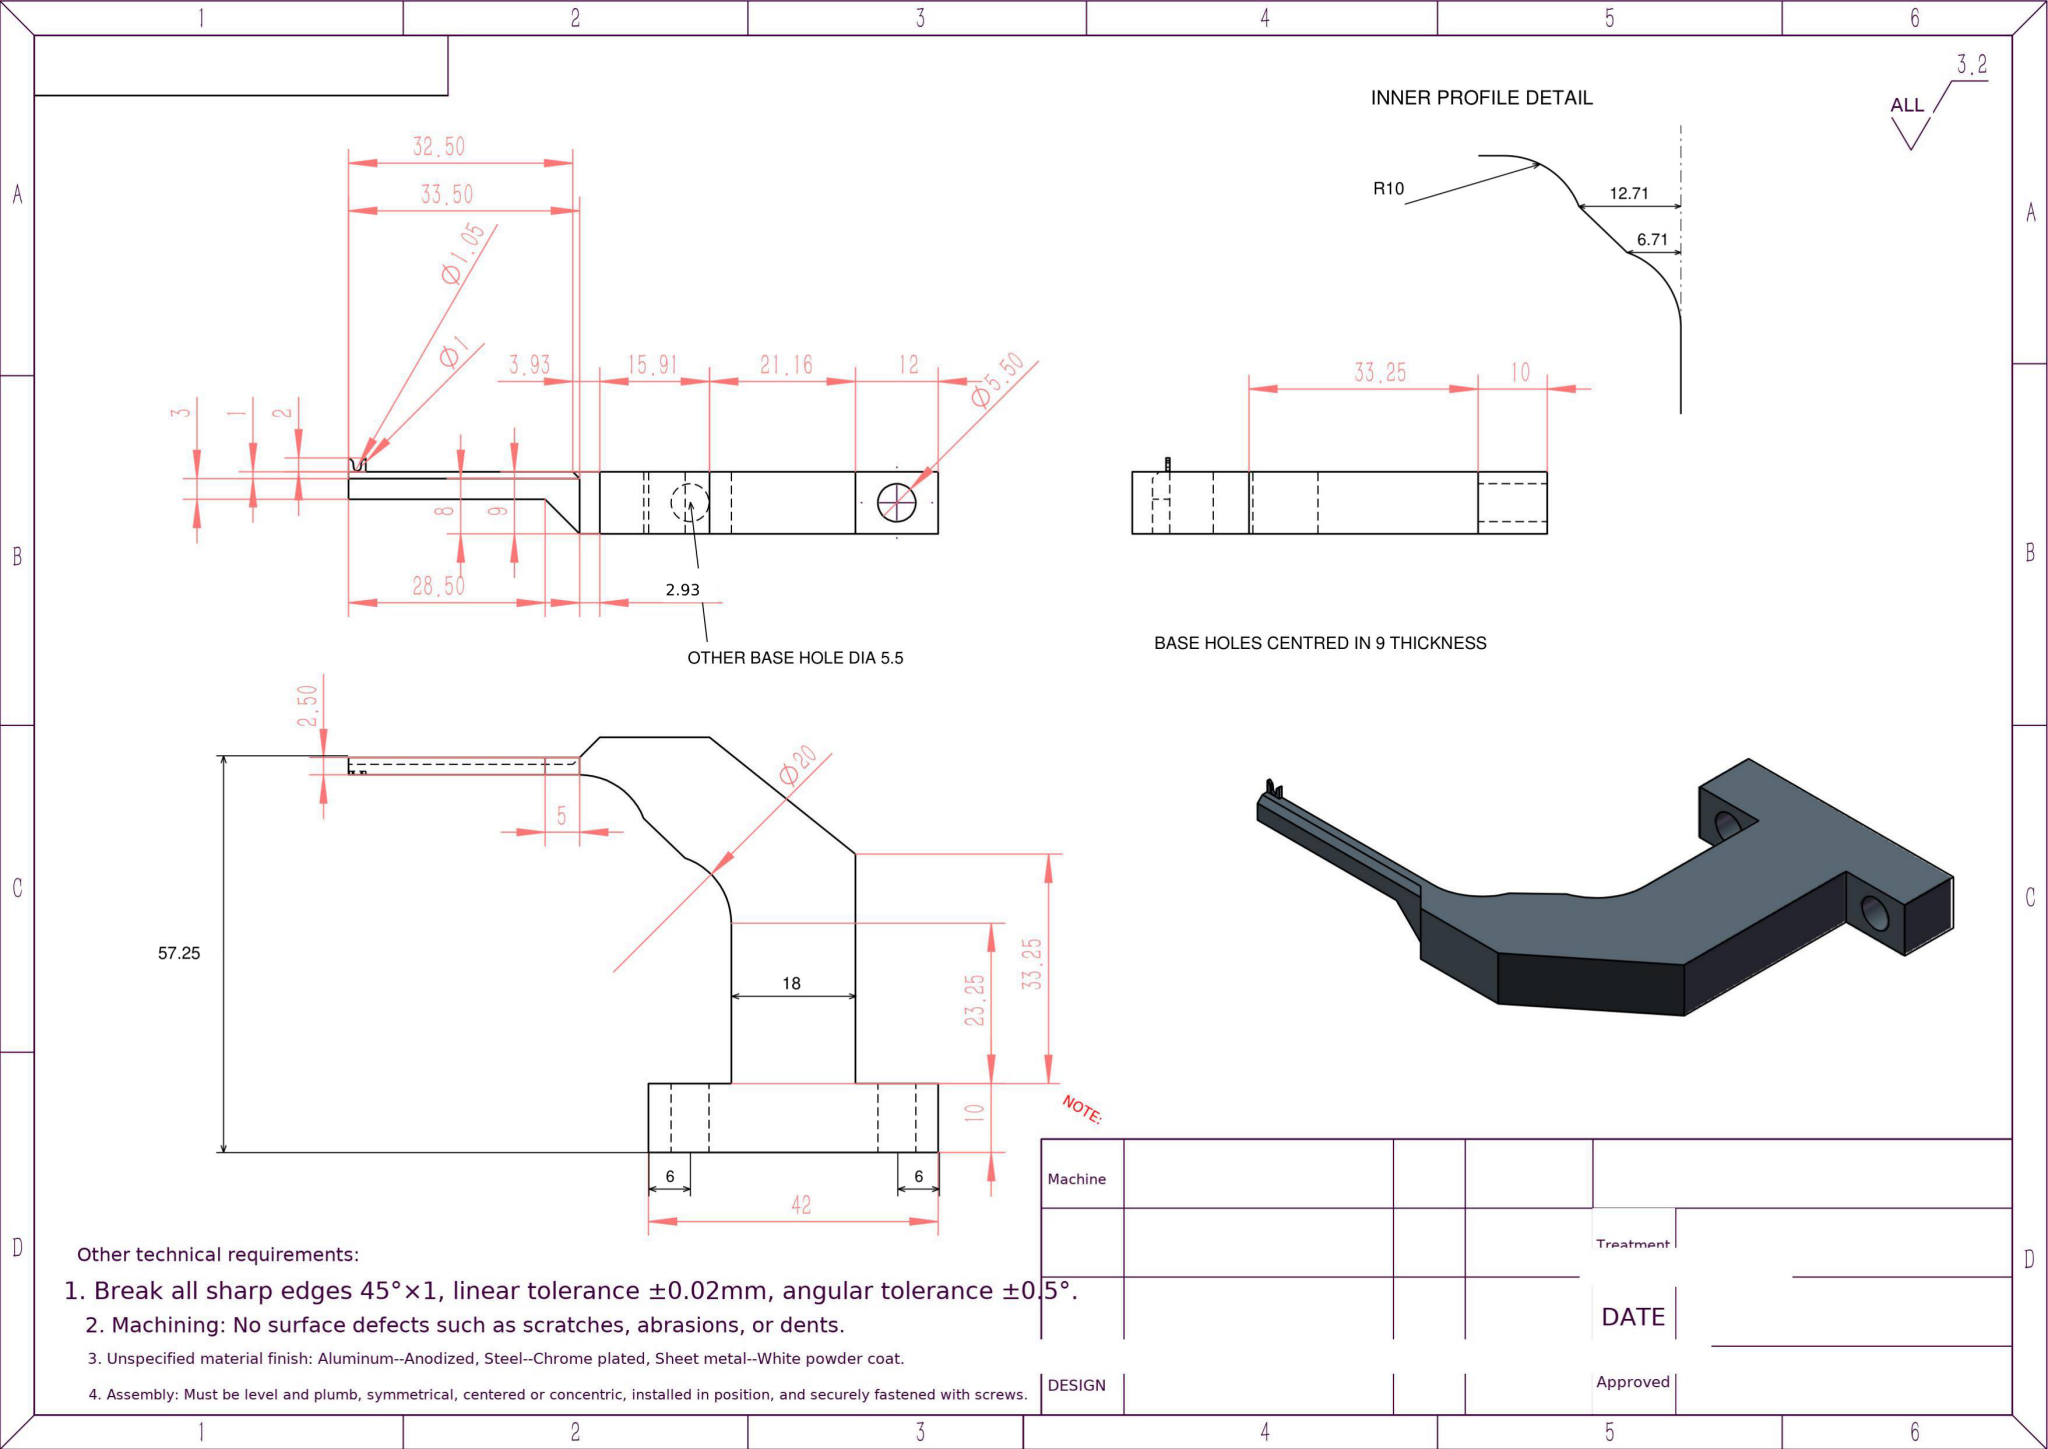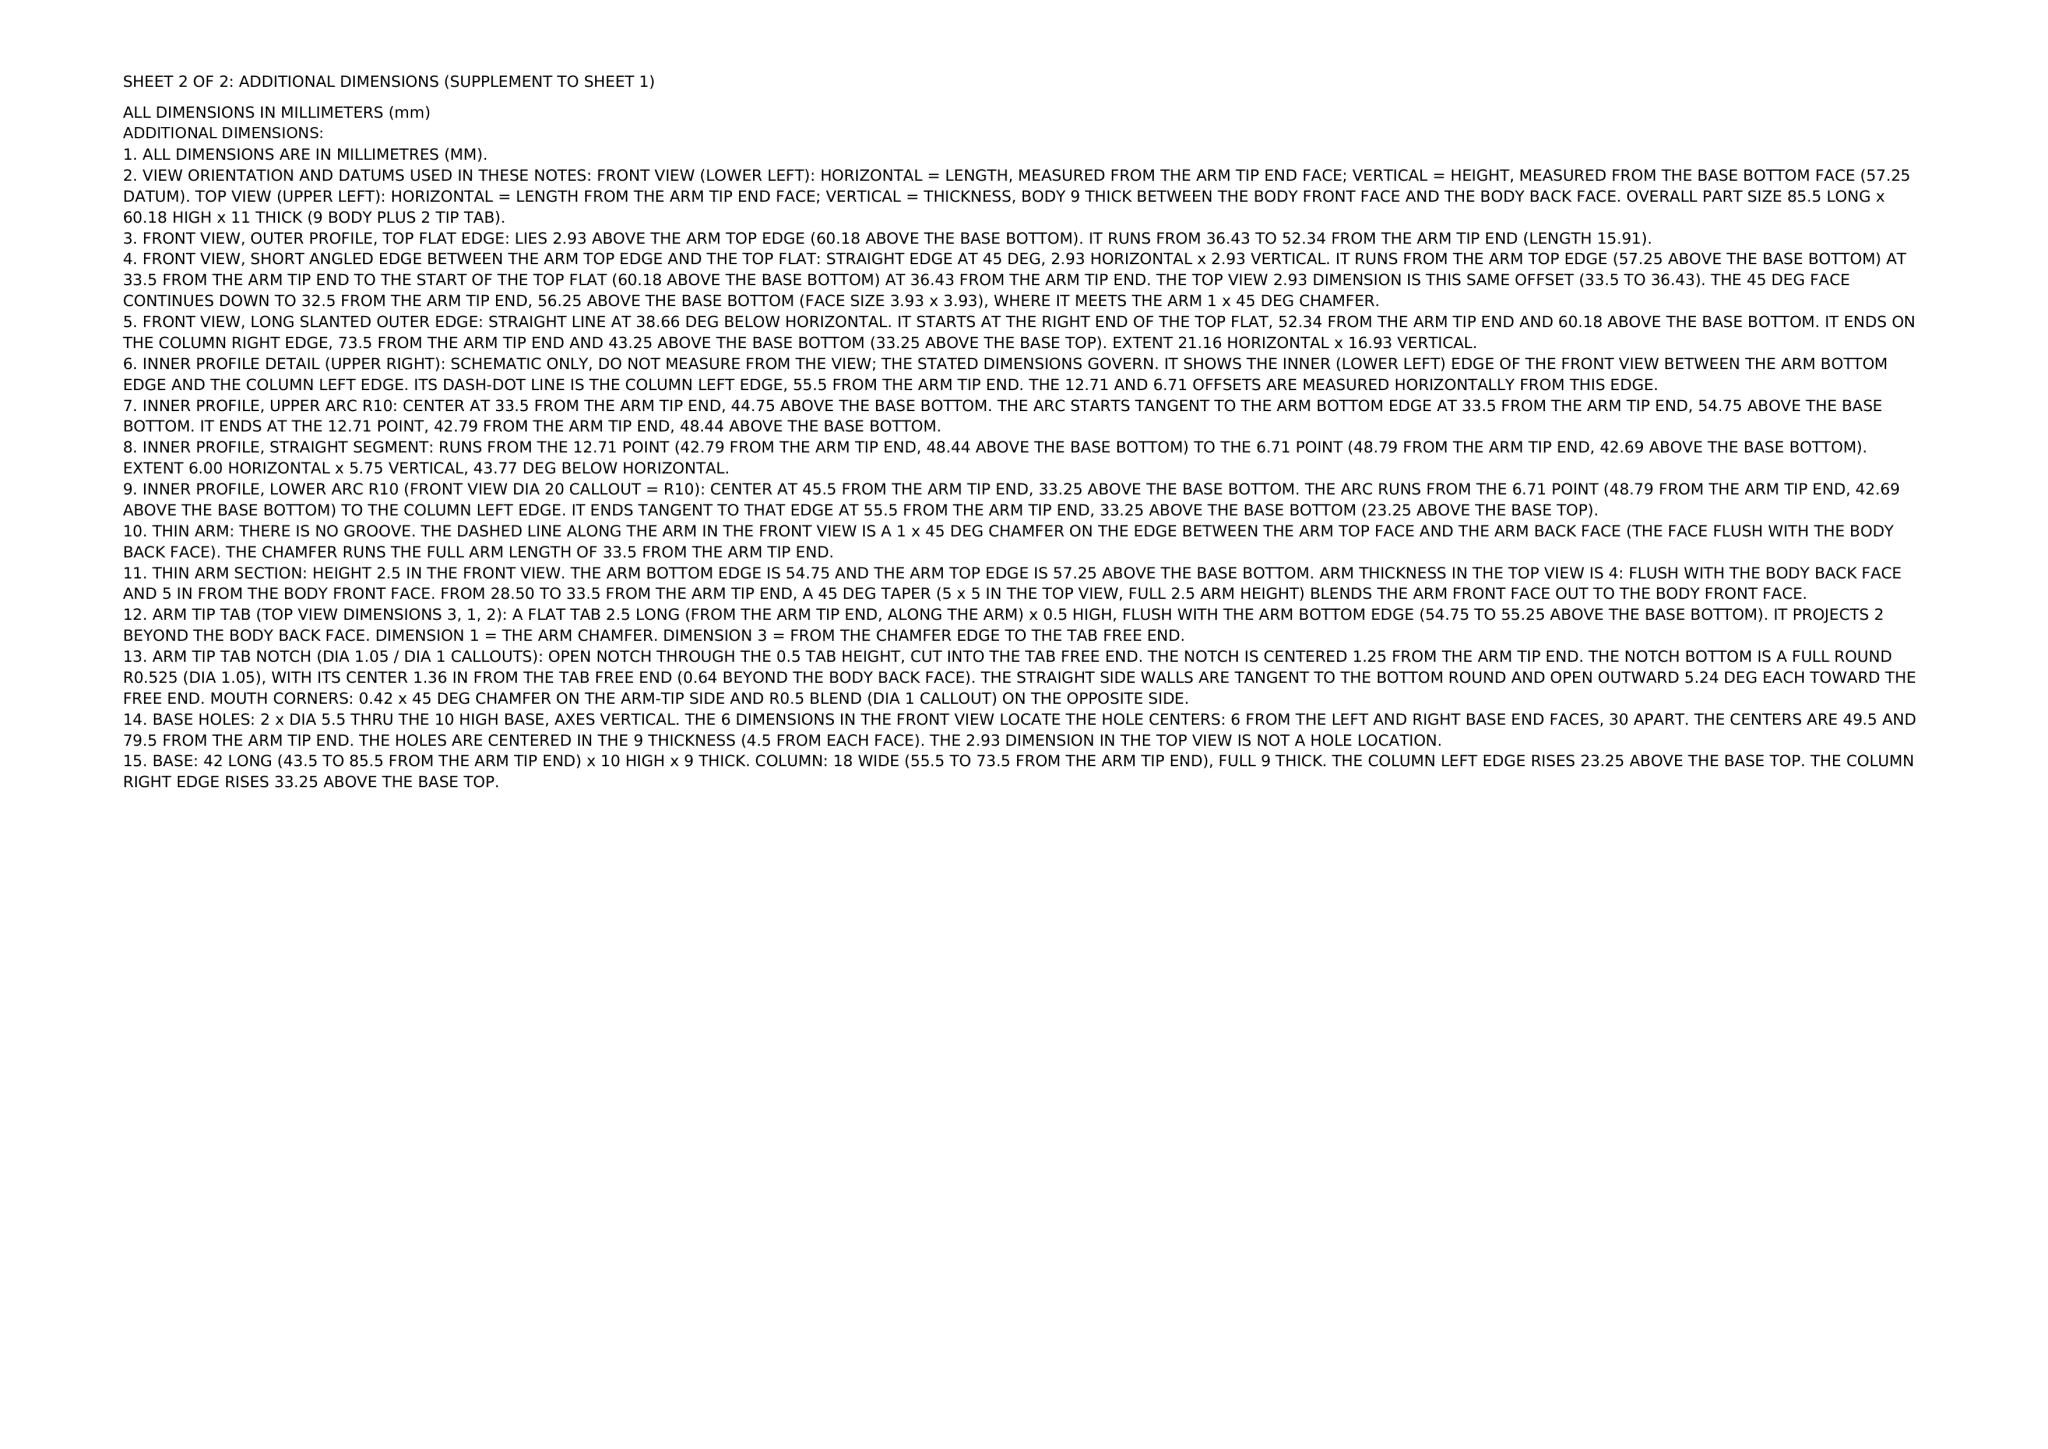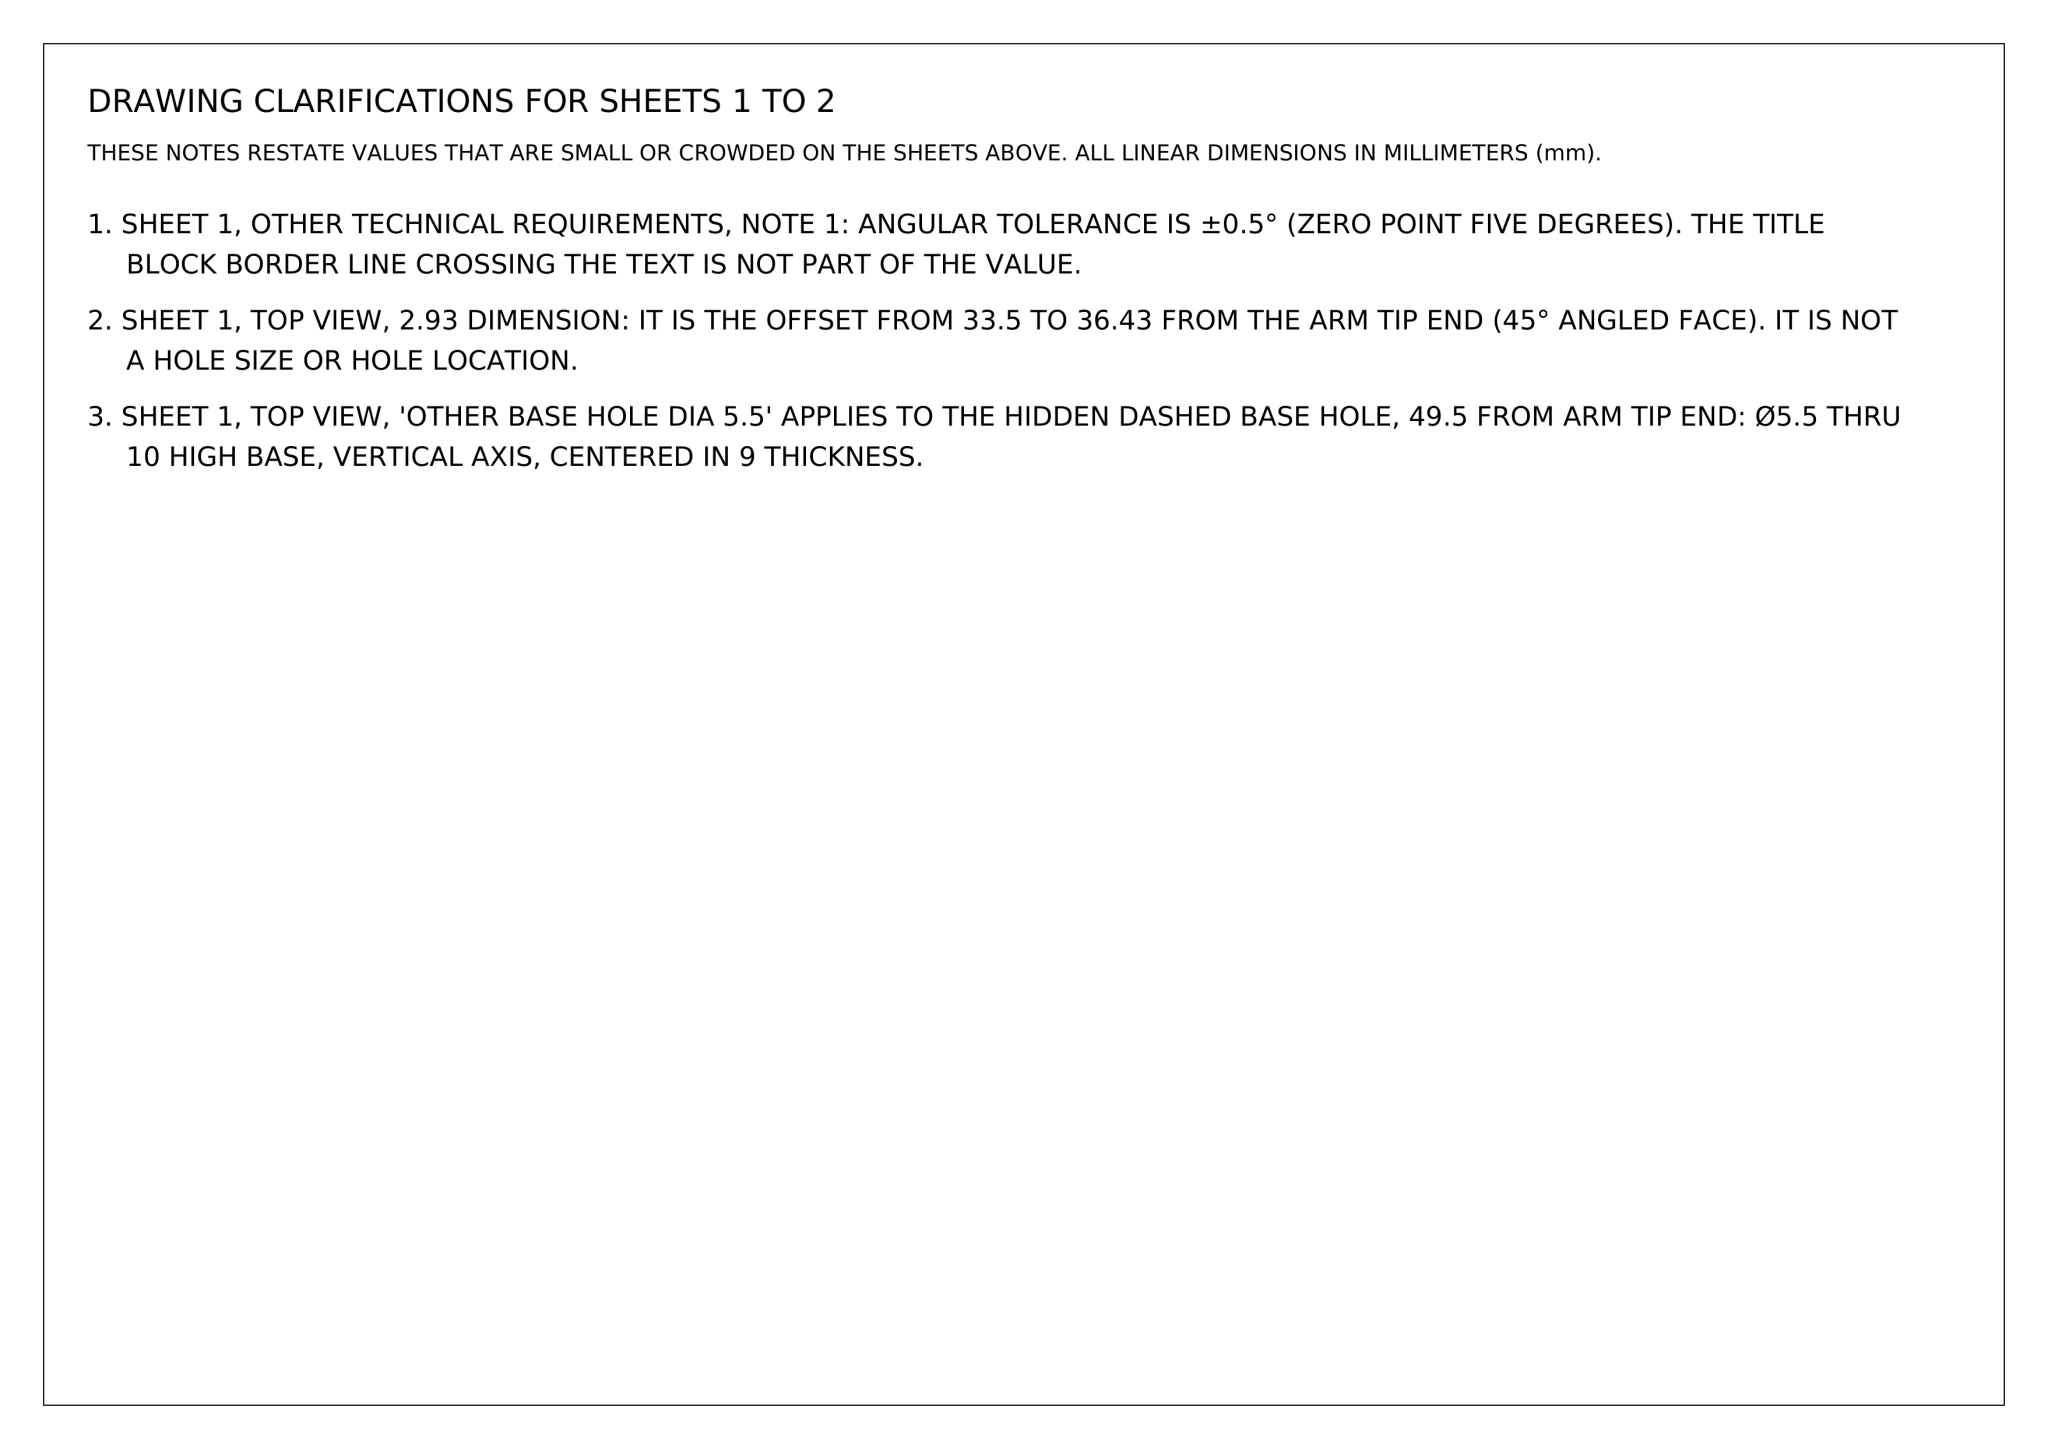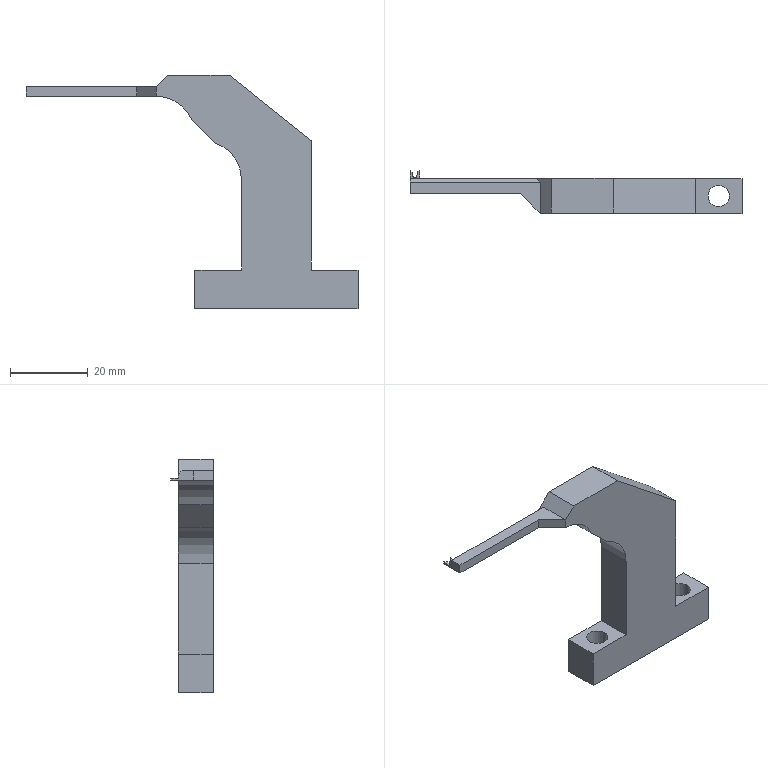Part | NX | mm | 1 solid | 36 faces | box 85.5 x 11 x 60.18 mm | volume 12732 mm3 | plane 27 | cylinder 9 | commonest cylinder face diameters 5.5 x4 1 x2 20 x2 1.05 x1